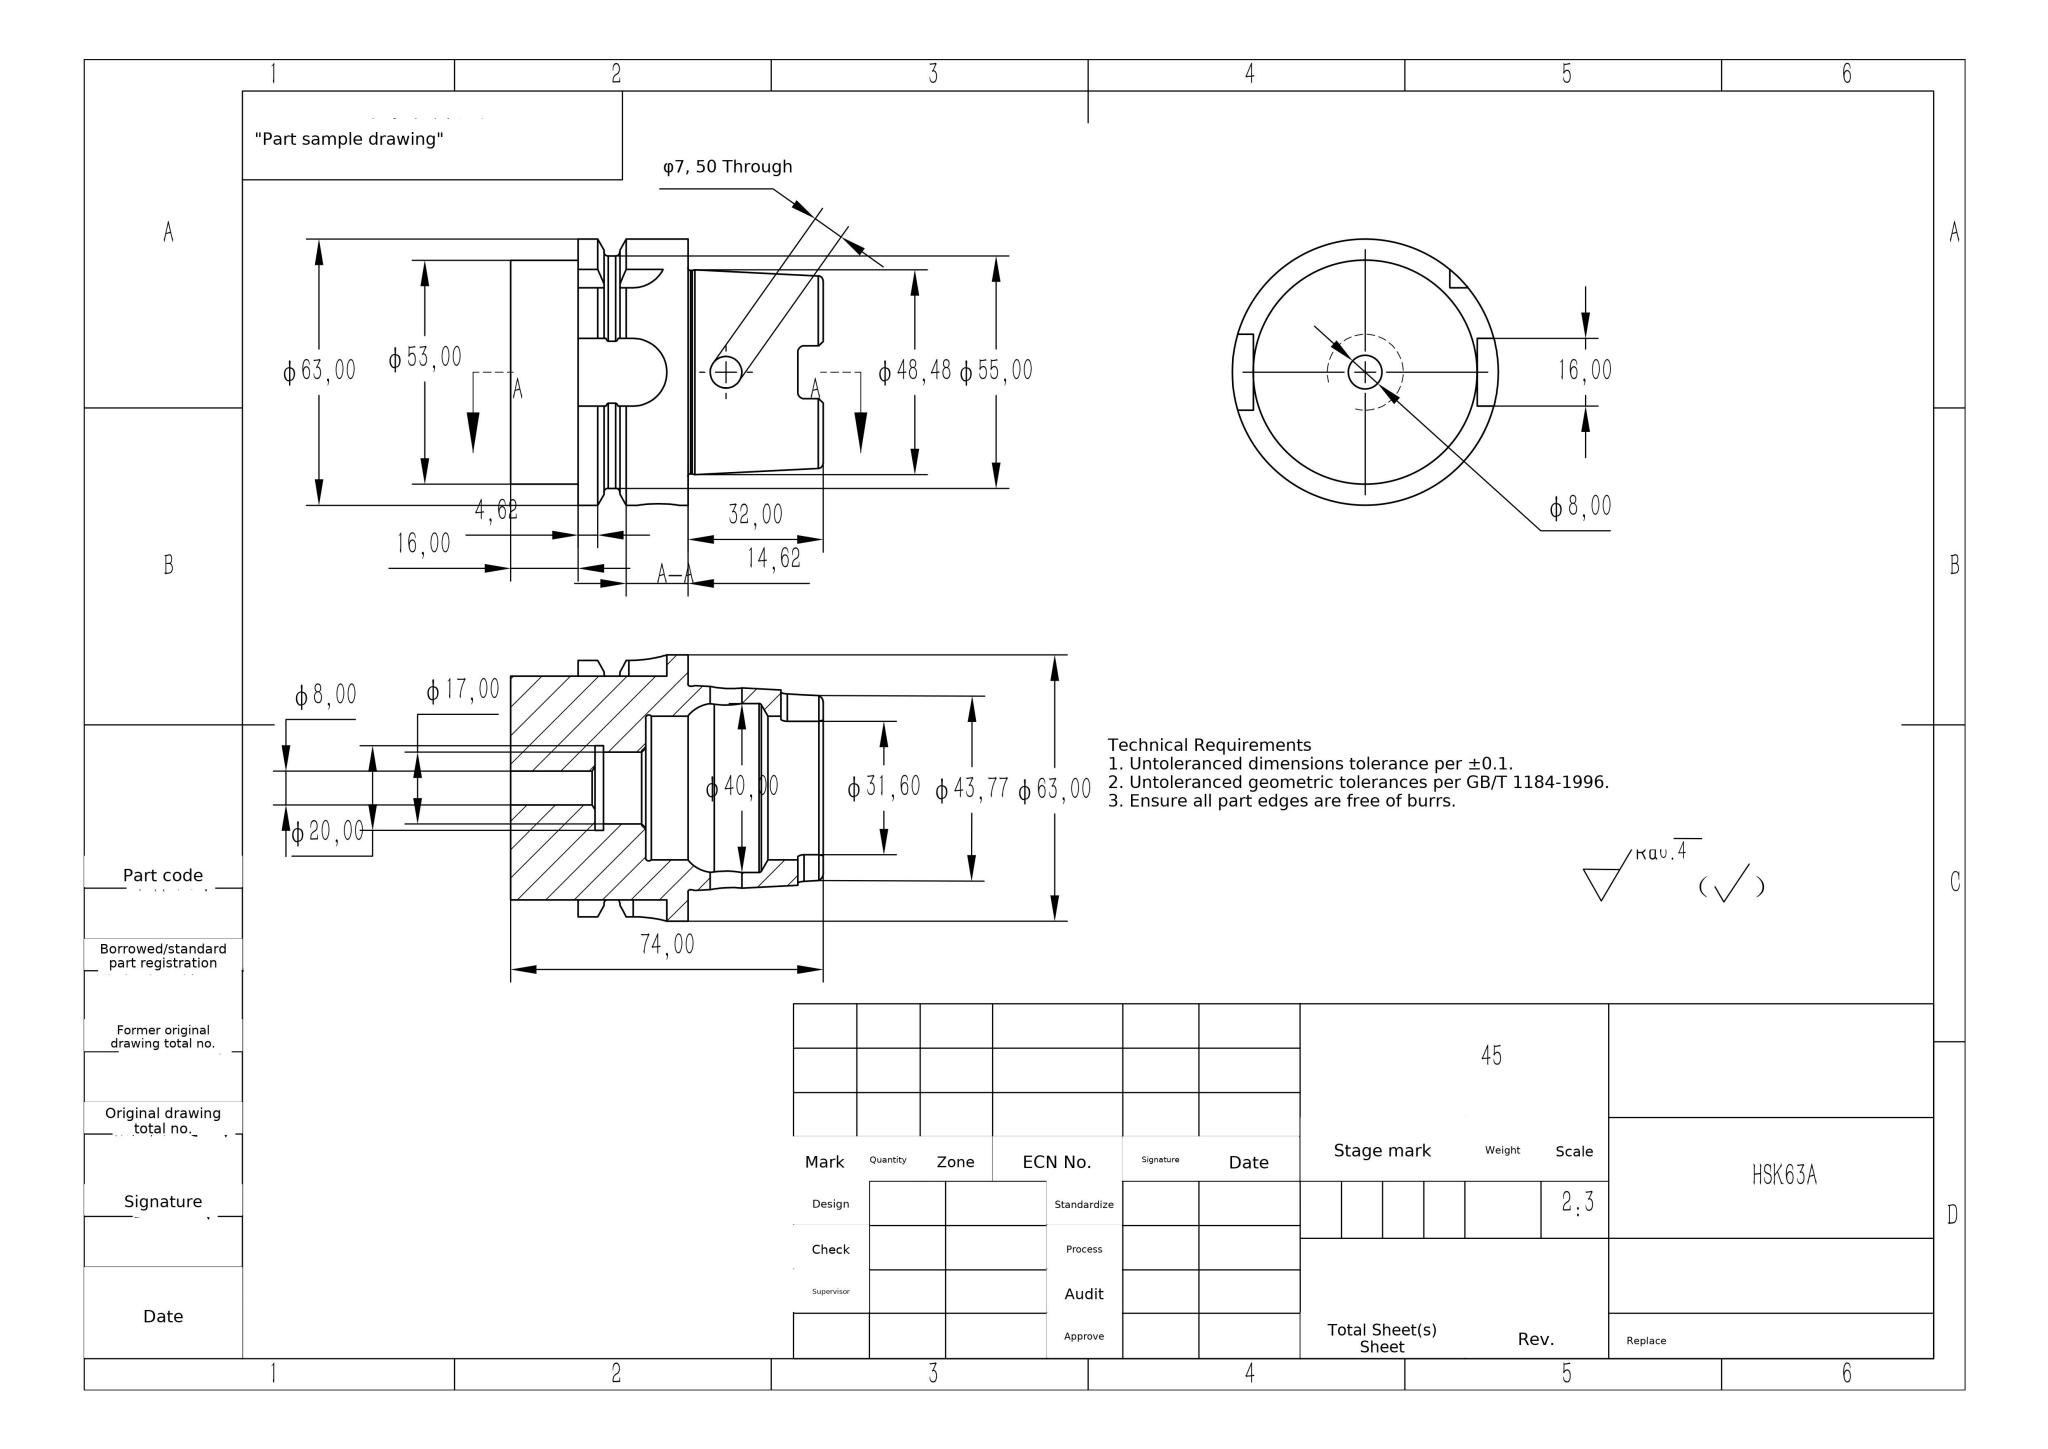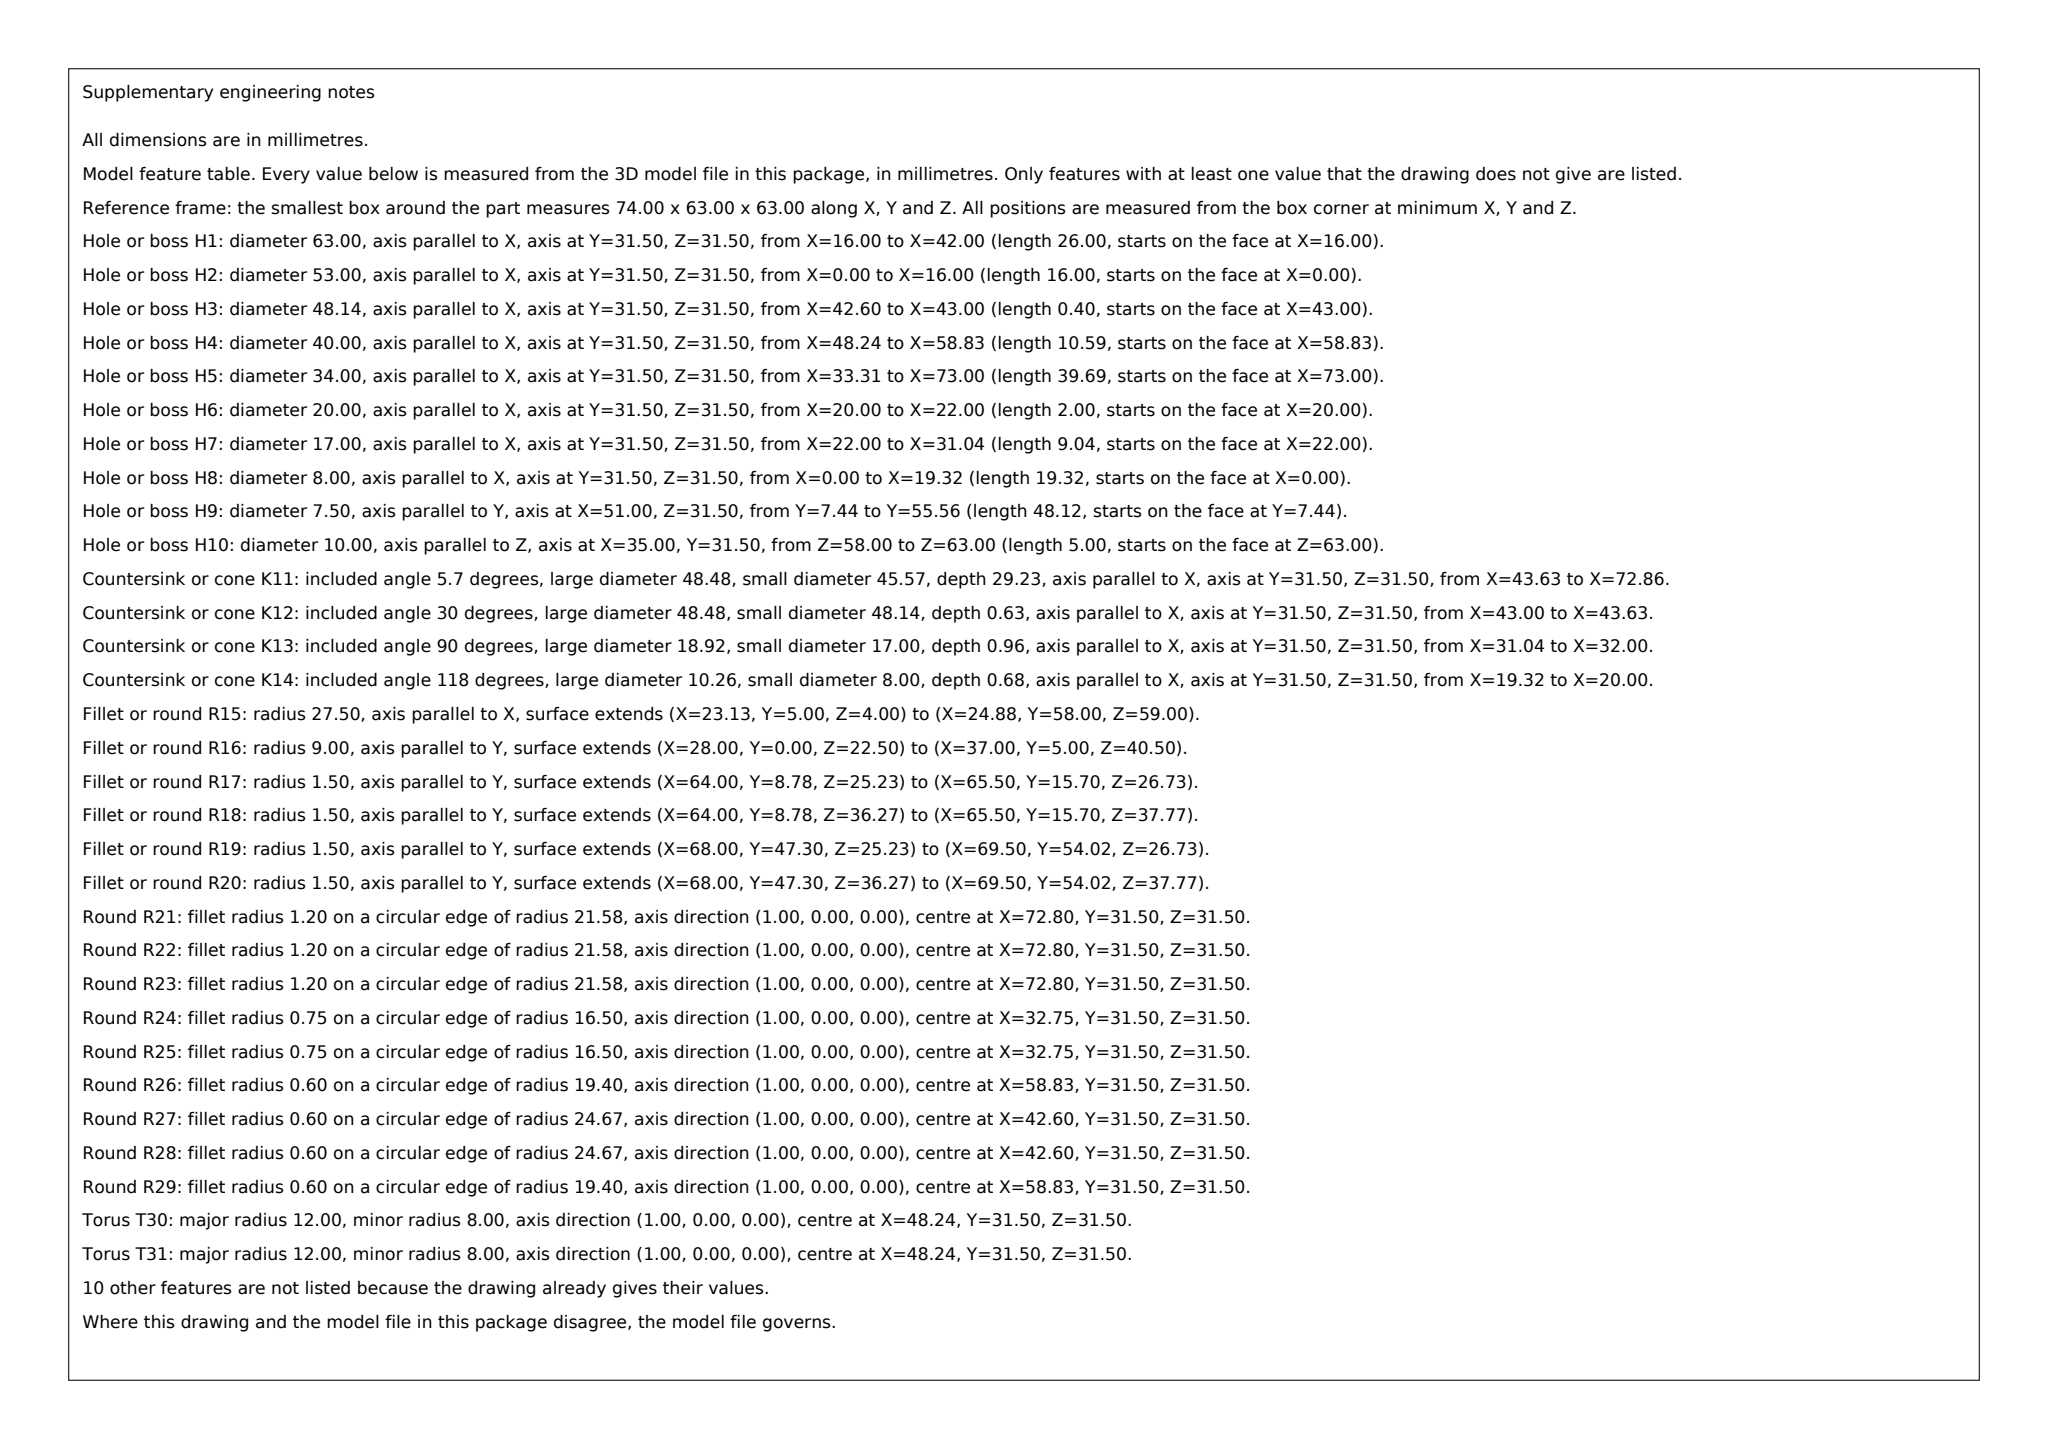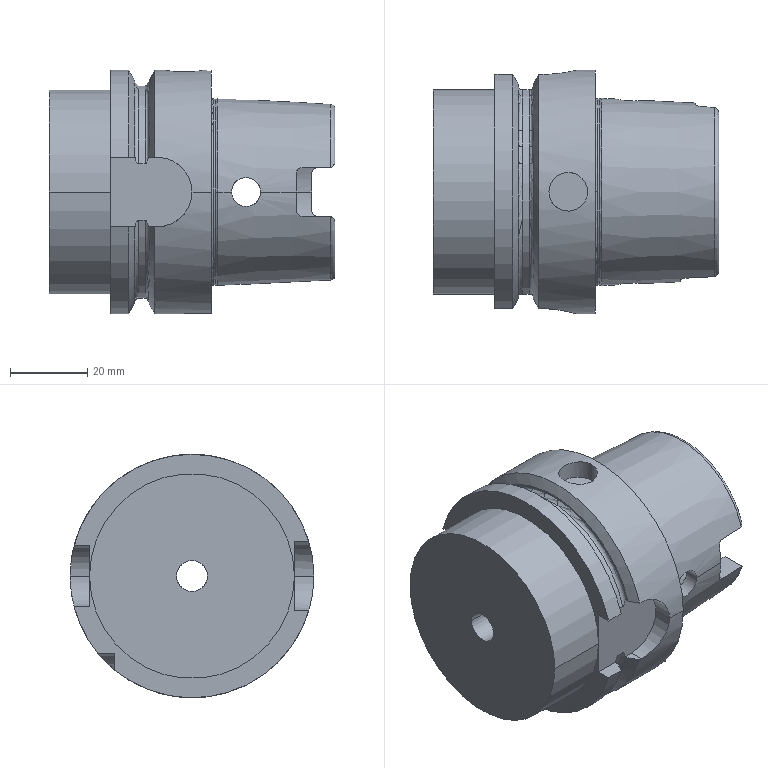Part | SolidWorks | mm | material 45 | 1 solid | 113 faces | box 74 x 63 x 63 mm | volume 116294 mm3 | plane 40 | cylinder 38 | cone 18 | torus 17 | commonest cylinder face diameters 63 x5 34 x4 7.5 x4 3 x4 16 x3 17 x2 8 x2 20 x2